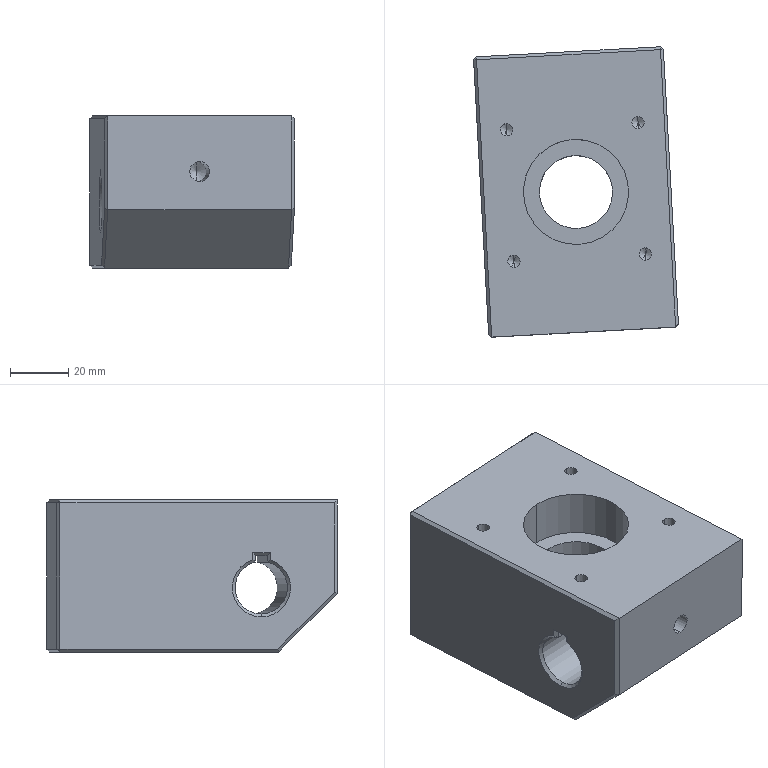Component | SolidWorks | BearingPressPartQ-1 | 1 solid | 65 faces | box 70.05 x 99.3 x 52 mm | volume 257549 mm3 | plane 33 | cylinder 17 | cone 15 | commonest cylinder face diameters 4.2 x8 8 x2 6.8 x2 36 x2 25 x2 18 x1
build123d program:
from build123d import *

# Parameters (mm, degrees)
SKETCH1_W             = 96
SKETCH1_H             = 65
BOSS_EXTRUDE1_DEPTH   = 52
CUT_EXTRUDE1_DEPTH    = 128.063
SKETCH3_R             = 12.5
CUT_EXTRUDE2_DEPTH    = 128.063
CHAMFER1_SIZE         = 20
SKETCH4_R             = 18
CUT_EXTRUDE3_DEPTH    = 16
M8_TAPPED_HOLE1_D     = 6.8
M8_TAPPED_HOLE1_DEPTH = 19.75
M8_TAPPED_HOLE1_TIP   = 2.043
M5_TAPPED_HOLE1_D     = 4.2
M5_TAPPED_HOLE1_DEPTH = 12.4
M5_TAPPED_HOLE1_TIP   = 1.262
CHAMFER2_SIZE         = 1
M8_TAPPED_HOLE2_D     = 8
M8_TAPPED_HOLE2_DEPTH = 19.75
M8_TAPPED_HOLE2_TIP   = 2.403


with BuildPart() as part:
    # Sketch1 → Boss-Extrude1 (new body)
    with BuildSketch(Plane.XY):
        with Locations((48, 32.5)):
            Rectangle(SKETCH1_W, SKETCH1_H)
    extrude(amount=BOSS_EXTRUDE1_DEPTH)

    # Sketch2 → Cut-Extrude1 (cut, through all)
    with BuildSketch(Plane.XZ):
        with BuildLine():
            Line((68, 21.225), (68, 19))
            Line((68, 19), (72, 19))
            Line((72, 19), (72, 21.225))
            ThreePointArc((72, 21.225), (70, 39), (68, 21.225))
        make_face()
    extrude(amount=-CUT_EXTRUDE1_DEPTH, mode=Mode.SUBTRACT)

    # Sketch3 → Cut-Extrude2 (cut, through all)
    with BuildSketch(Plane.XY.offset(52)):
        with Locations((48, 32.5)):
            Circle(SKETCH3_R)
    extrude(amount=-CUT_EXTRUDE2_DEPTH, mode=Mode.SUBTRACT)

    # Chamfer1
    chamfer1_edges = [part.edges().sort_by_distance(p)[0] for p in [
        (96, 32.5, 52),
    ]]
    chamfer(chamfer1_edges, length=CHAMFER1_SIZE)

    # Sketch4 → Cut-Extrude3 (cut)
    with BuildSketch(Plane(origin=(0, 0, 0), x_dir=(-1, 0, 0), z_dir=(0, 0, -1))):
        with Locations((-48, 32.5)):
            Circle(SKETCH4_R)
    extrude(amount=-CUT_EXTRUDE3_DEPTH, mode=Mode.SUBTRACT)

    # M8 Tapped Hole1
    with Locations(Plane(origin=(96, 0, 0), x_dir=(0, 0, -1), z_dir=(1, 0, 0))):
        with Locations((-19, 32.5)):
            Hole(M8_TAPPED_HOLE1_D / 2, depth=M8_TAPPED_HOLE1_DEPTH)
            with Locations((0, 0, -(M8_TAPPED_HOLE1_DEPTH + M8_TAPPED_HOLE1_TIP / 2))):  # 118° drill point
                Cone(0, M8_TAPPED_HOLE1_D / 2, M8_TAPPED_HOLE1_TIP, mode=Mode.SUBTRACT)

    # M5 Tapped Hole1
    with Locations(Plane(origin=(0, 0, 0), x_dir=(-1, 0, 0), z_dir=(0, 0, -1))):
        with Locations((-25.5, 10), (-70.5, 10), (-70.5, 55), (-25.5, 55)):
            Hole(M5_TAPPED_HOLE1_D / 2, depth=M5_TAPPED_HOLE1_DEPTH)
            with Locations((0, 0, -(M5_TAPPED_HOLE1_DEPTH + M5_TAPPED_HOLE1_TIP / 2))):  # 118° drill point
                Cone(0, M5_TAPPED_HOLE1_D / 2, M5_TAPPED_HOLE1_TIP, mode=Mode.SUBTRACT)

    # Chamfer2
    chamfer2_edges = [part.edges().sort_by_distance(p)[0] for p in [
        (70, 65, 19),
        (68, 65, 20.113),
        (70, 65, 39),
        (72, 65, 20.113),
        (70, 0, 19),
        (72, 0, 20.113),
        (70, 0, 39),
        (68, 0, 20.113),
        (38, 65, 52),
        (96, 65, 16),
        (86, 65, 42),
        (96, 0, 16),
        (86, 0, 42),
        (0, 32.5, 52),
        (48, 65, 0),
        (48, 0, 0),
        (0, 32.5, 0),
        (38, 0, 52),
        (0, 65, 26),
        (0, 0, 26),
    ]]
    chamfer(chamfer2_edges, length=CHAMFER2_SIZE)

    # M8 Tapped Hole2
    with Locations(Plane.XY.offset(52)):
        with Locations((16, 32.5)):
            Hole(M8_TAPPED_HOLE2_D / 2, depth=M8_TAPPED_HOLE2_DEPTH)
            with Locations((0, 0, -(M8_TAPPED_HOLE2_DEPTH + M8_TAPPED_HOLE2_TIP / 2))):  # 118° drill point
                Cone(0, M8_TAPPED_HOLE2_D / 2, M8_TAPPED_HOLE2_TIP, mode=Mode.SUBTRACT)


solid = part.part

# Placed as in the assembly
solid = solid.moved(Location((477.501, 177.67, -187.818), (-180, 0, 86.863)))